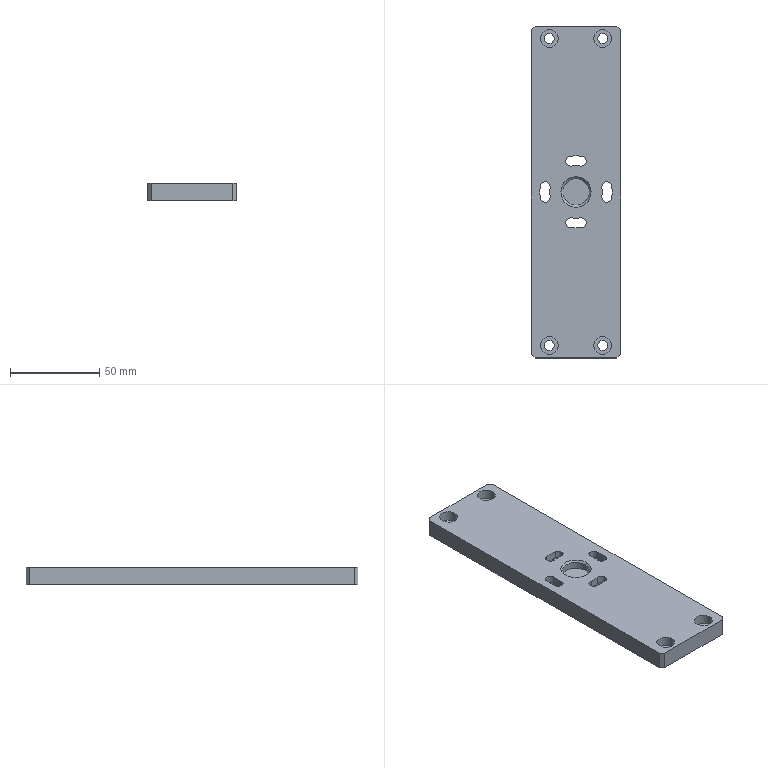CAM job | Mastercam | mm | 15 operations | part box 50 x 186.4 x 10
1. Drill/Counterbore | 2 - 6定位倒角
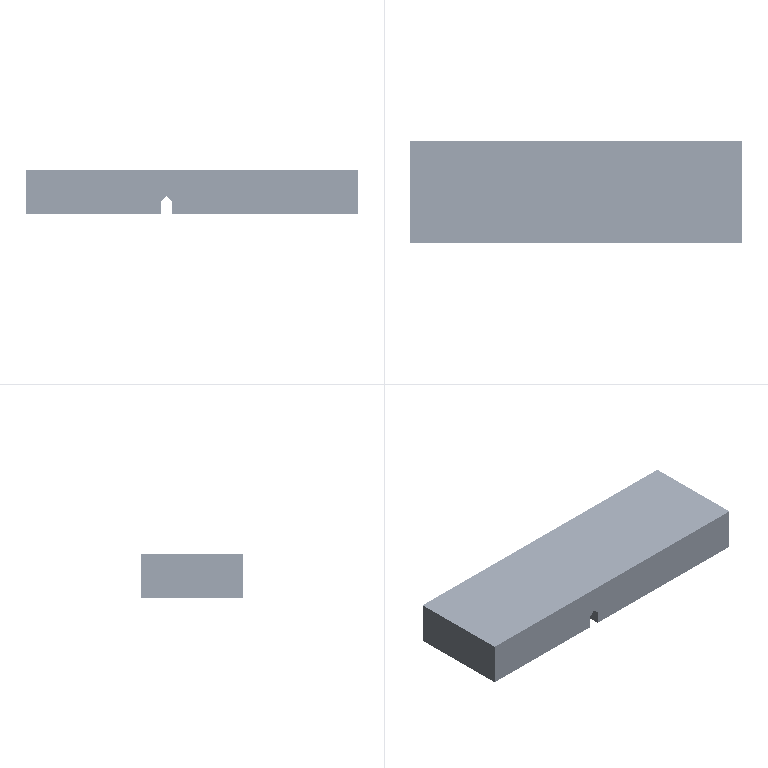2. Peck Drill | 16 - 5.5 钻头
3. Contour (Ramp) | 5 - 6 C平底刀
4. Contour (Ramp) | 7 - 4 C平底刀
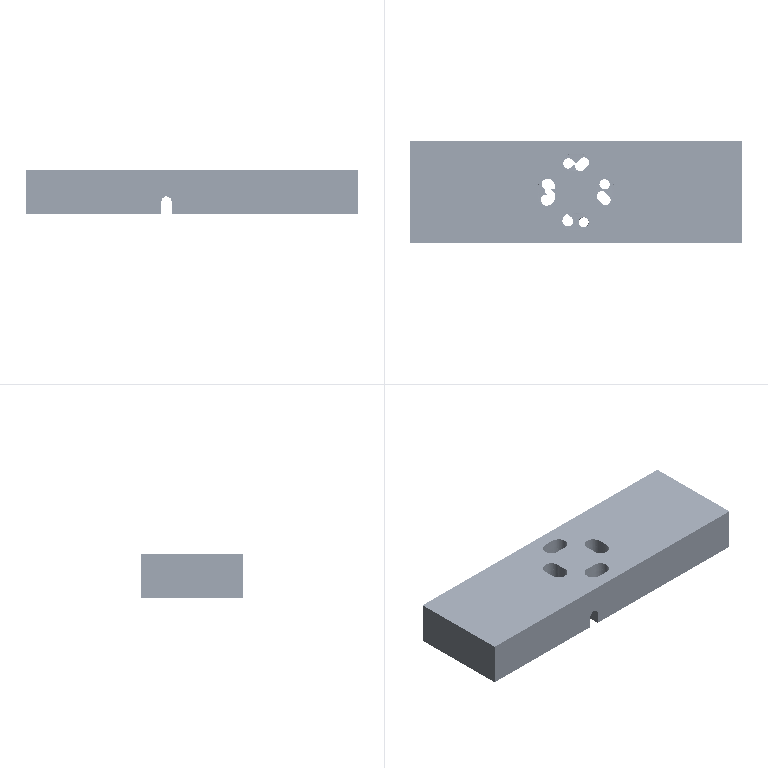5. Contour (2D) | 5 - 6 C平底刀
6. Contour (2D) | 7 - 4 C平底刀
7. Contour (Ramp) | 3 - 8 C 平底刀
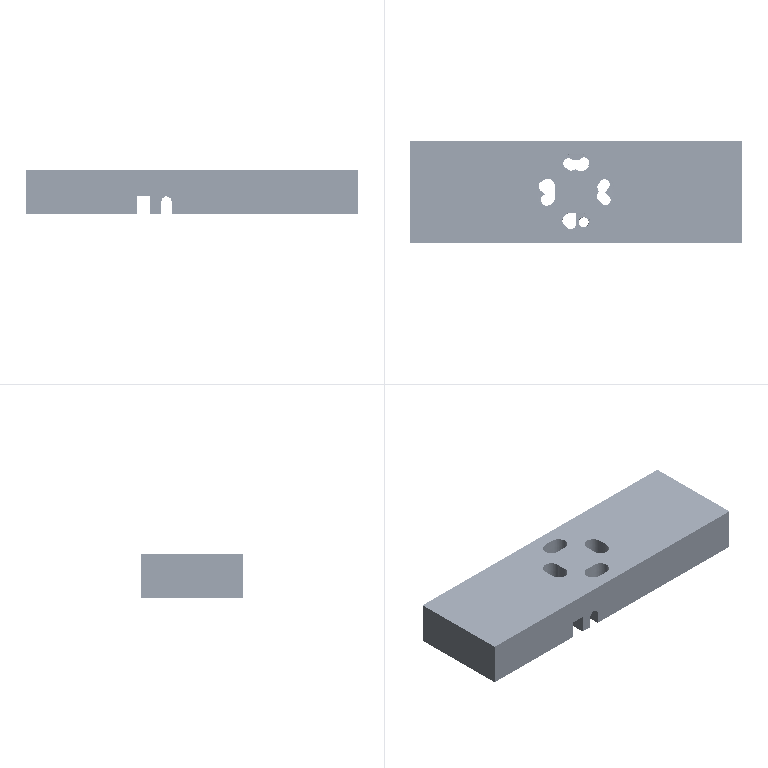8. Contour (2D) | 4 - 8 J平底刀
9. Model Chamfer | 2 - 6定位倒角
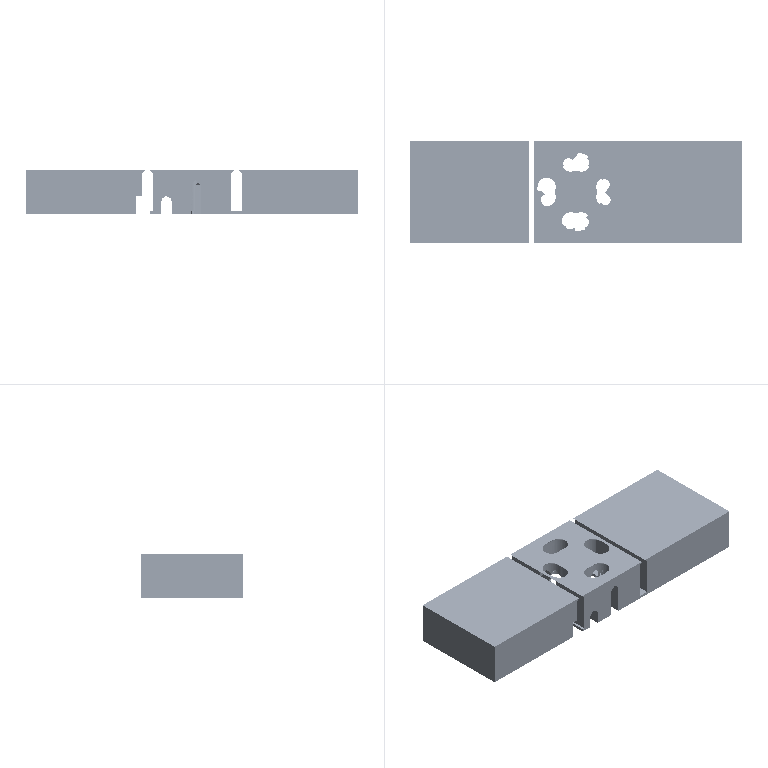10. Contour (2D) | 4 - 8 J平底刀
11. Helix Bore | 5 - 6 C平底刀
12. Helix Bore | 9 - 10C 平底刀
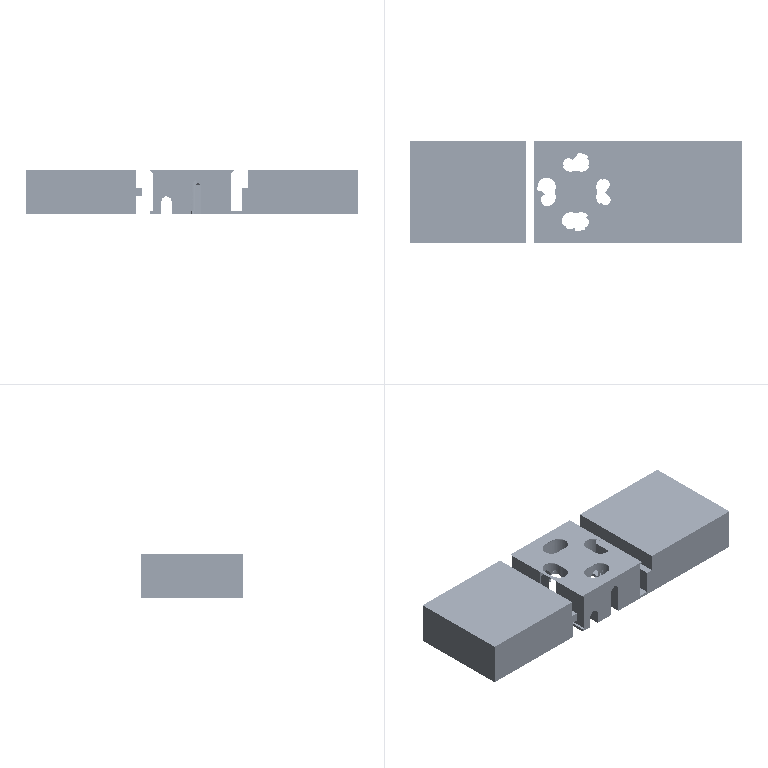13. Circle Mill | 10 - 10 J平底刀
14. Model Chamfer | 2 - 6定位倒角
15. Contour (2D chamfer) | 2 - 6定位倒角